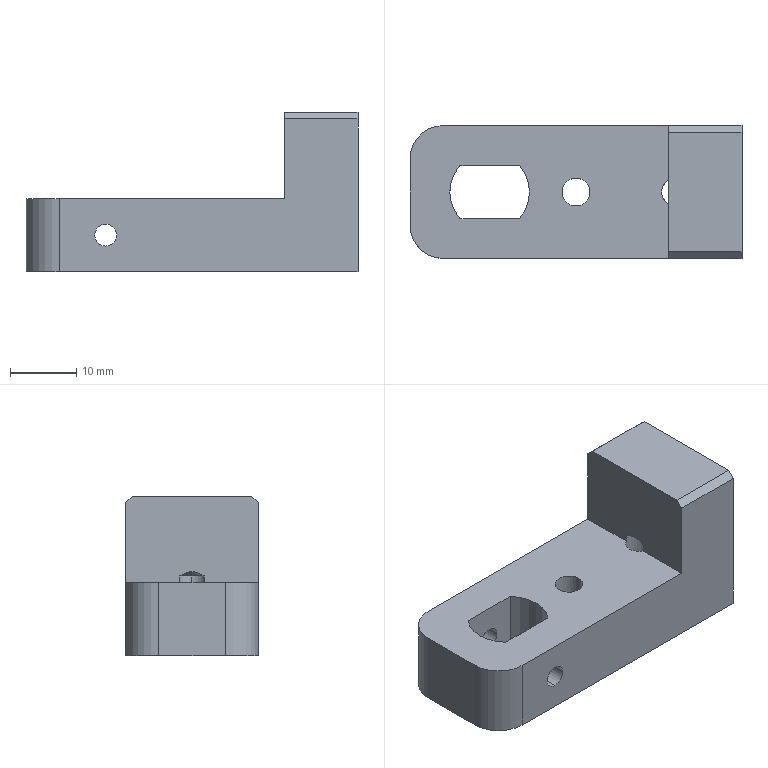Component | SolidWorks | TensioningWheel-2-1_XT-1-20-2-1 | 1 solid | 27 faces | box 50 x 20 x 24 mm | volume 12336 mm3 | cylinder 13 | plane 12 | cone 2 | commonest cylinder face diameters 3.3 x4 4.2 x4 12 x3 10 x2
build123d program:
from build123d import *

# Parameters (mm, degrees)
SKETCH1_W             = 50
SKETCH1_H             = 20
BOSS_EXTRUDE1_DEPTH   = 11
SKETCH7_W             = 11
SKETCH7_H             = 20
BOSS_EXTRUDE3_DEPTH   = 13
M5_TAPPED_HOLE1_D     = 4.2
M5_TAPPED_HOLE1_DEPTH = 12
M5_TAPPED_HOLE1_TIP   = 1.262
FILLET1_R             = 5
M4_TAPPED_HOLE1_D     = 3.3
CHAMFER1_SIZE         = 1


with BuildPart() as part:
    # Sketch1 → Boss-Extrude1 (new body)
    with BuildSketch(Plane.XY):
        with Locations((25, -10)):
            Rectangle(SKETCH1_W, SKETCH1_H)
        with BuildLine():
            Line((7.528, -6), (16.472, -6))
            ThreePointArc((16.472, -6), (18, -10), (16.472, -14))
            Line((16.472, -14), (7.528, -14))
            ThreePointArc((7.528, -14), (6, -10), (7.528, -6))
        make_face(mode=Mode.SUBTRACT)
    extrude(amount=BOSS_EXTRUDE1_DEPTH)

    # Sketch7 → Boss-Extrude3 (add)
    with BuildSketch(Plane.XY.offset(11)):
        with Locations((44.5, -10)):
            Rectangle(SKETCH7_W, SKETCH7_H)
    extrude(amount=BOSS_EXTRUDE3_DEPTH)

    # M5 Tapped Hole1
    with Locations(Plane(origin=(0, 0, 0), x_dir=(-1, 0, 0), z_dir=(0, 0, -1))):
        with Locations((-40, -10), (-25, -10)):
            Hole(M5_TAPPED_HOLE1_D / 2, depth=M5_TAPPED_HOLE1_DEPTH)
            with Locations((0, 0, -(M5_TAPPED_HOLE1_DEPTH + M5_TAPPED_HOLE1_TIP / 2))):  # 118° drill point
                Cone(0, M5_TAPPED_HOLE1_D / 2, M5_TAPPED_HOLE1_TIP, mode=Mode.SUBTRACT)

    # Fillet1
    fillet1_edges = [part.edges().sort_by_distance(p)[0] for p in [
        (0, -20, 5.5),
        (0, 0, 5.5),
    ]]
    fillet(fillet1_edges, radius=FILLET1_R)

    # M4 Tapped Hole1 (through all)
    with Locations(Plane(origin=(0, 0, 0), x_dir=(1, 0, 0), z_dir=(0, 1, 0))):
        with Locations((12, -5.5)):
            Hole(M4_TAPPED_HOLE1_D / 2)

    # Chamfer1
    chamfer1_edges = [part.edges().sort_by_distance(p)[0] for p in [
        (44.5, -20, 24),
        (44.5, 0, 24),
    ]]
    chamfer(chamfer1_edges, length=CHAMFER1_SIZE)


solid = part.part

# Placed as in the assembly
solid = solid.moved(Location((526.036, -108.615, -151), (0, 0, 0)))
STEP:
#1=CARTESIAN_POINT('',(21.183,-5.064,-5.793));
#2=VERTEX_POINT('',#1);
#3=CARTESIAN_POINT('',(21.183,-5.064,-5.663));
#4=VERTEX_POINT('',#3);
#5=CARTESIAN_POINT('',(21.183,-5.064,-5.728));
#6=DIRECTION('',(0.,1.,0.));
#7=DIRECTION('',(0.,0.,1.));
#8=AXIS2_PLACEMENT_3D('',#5,#6,#7);
#9=CIRCLE('',#8,0.06496);
#10=EDGE_CURVE('',#2,#4,#9,.T.);
#11=ORIENTED_EDGE('',*,*,#10,.F.);
#12=CARTESIAN_POINT('',(21.183,-4.827,-5.793));
#13=VERTEX_POINT('',#12);
#14=CARTESIAN_POINT('',(21.183,-4.276,-5.793));
#15=DIRECTION('',(0.,1.,0.));
#16=VECTOR('',#15,39.37);
#17=LINE('',#14,#16);
#18=EDGE_CURVE('',#2,#13,#17,.T.);
#19=ORIENTED_EDGE('',*,*,#18,.T.);
#20=CARTESIAN_POINT('',(21.183,-4.827,-5.663));
#21=VERTEX_POINT('',#20);
#22=CARTESIAN_POINT('',(21.183,-4.827,-5.728));
#23=DIRECTION('',(0.,1.,0.));
#24=DIRECTION('',(0.,0.,1.));
#25=AXIS2_PLACEMENT_3D('',#22,#23,#24);
#26=CIRCLE('',#25,0.06496);
#27=EDGE_CURVE('',#13,#21,#26,.T.);
#28=ORIENTED_EDGE('',*,*,#27,.T.);
#29=CARTESIAN_POINT('',(21.183,-4.276,-5.663));
#30=DIRECTION('',(0.,1.,0.));
#31=VECTOR('',#30,39.37);
#32=LINE('',#29,#31);
#33=EDGE_CURVE('',#4,#21,#32,.T.);
#34=ORIENTED_EDGE('',*,*,#33,.F.);
#35=EDGE_LOOP('',(#11,#19,#28,#34));
#36=FACE_OUTER_BOUND('',#35,.T.);
#37=CARTESIAN_POINT('',(21.183,-4.276,-5.728));
#38=DIRECTION('',(0.,1.,0.));
#39=DIRECTION('',(0.,0.,1.));
#40=AXIS2_PLACEMENT_3D('',#37,#38,#39);
#41=CYLINDRICAL_SURFACE('',#40,0.06496);
#42=ADVANCED_FACE('',(#36),#41,.F.);
#43=CARTESIAN_POINT('',(21.183,-4.512,-5.663));
#44=VERTEX_POINT('',#43);
#45=CARTESIAN_POINT('',(21.183,-4.512,-5.793));
#46=VERTEX_POINT('',#45);
#47=CARTESIAN_POINT('',(21.183,-4.512,-5.728));
#48=DIRECTION('',(0.,-1.,0.));
#49=DIRECTION('',(0.,0.,-1.));
#50=AXIS2_PLACEMENT_3D('',#47,#48,#49);
#51=CIRCLE('',#50,0.06496);
#52=EDGE_CURVE('',#44,#46,#51,.T.);
#53=ORIENTED_EDGE('',*,*,#52,.T.);
#54=CARTESIAN_POINT('',(21.183,-4.276,-5.793));
#55=VERTEX_POINT('',#54);
#56=CARTESIAN_POINT('',(21.183,-4.276,-5.793));
#57=DIRECTION('',(0.,1.,0.));
#58=VECTOR('',#57,39.37);
#59=LINE('',#56,#58);
#60=EDGE_CURVE('',#46,#55,#59,.T.);
#61=ORIENTED_EDGE('',*,*,#60,.T.);
#62=CARTESIAN_POINT('',(21.183,-4.276,-5.663));
#63=VERTEX_POINT('',#62);
#64=CARTESIAN_POINT('',(21.183,-4.276,-5.728));
#65=DIRECTION('',(0.,1.,0.));
#66=DIRECTION('',(0.,0.,1.));
#67=AXIS2_PLACEMENT_3D('',#64,#65,#66);
#68=CIRCLE('',#67,0.06496);
#69=EDGE_CURVE('',#55,#63,#68,.T.);
#70=ORIENTED_EDGE('',*,*,#69,.T.);
#71=CARTESIAN_POINT('',(21.183,-4.276,-5.663));
#72=DIRECTION('',(0.,1.,0.));
#73=VECTOR('',#72,39.37);
#74=LINE('',#71,#73);
#75=EDGE_CURVE('',#44,#63,#74,.T.);
#76=ORIENTED_EDGE('',*,*,#75,.F.);
#77=EDGE_LOOP('',(#53,#61,#70,#76));
#78=FACE_OUTER_BOUND('',#77,.T.);
#79=CARTESIAN_POINT('',(21.183,-4.276,-5.728));
#80=DIRECTION('',(0.,1.,0.));
#81=DIRECTION('',(0.,0.,1.));
#82=AXIS2_PLACEMENT_3D('',#79,#80,#81);
#83=CYLINDRICAL_SURFACE('',#82,0.06496);
#84=ADVANCED_FACE('',(#78),#83,.F.);
#85=CARTESIAN_POINT('',(22.285,-4.67,-5.423));
#86=VERTEX_POINT('',#85);
#87=CARTESIAN_POINT('',(22.246,-4.67,-5.446));
#88=VERTEX_POINT('',#87);
#89=CARTESIAN_POINT('',(22.202,-4.67,-5.472));
#90=DIRECTION('',(-0.8572,0.,-0.515));
#91=VECTOR('',#90,39.37);
#92=LINE('',#89,#91);
#93=EDGE_CURVE('',#86,#88,#92,.T.);
#94=ORIENTED_EDGE('',*,*,#93,.F.);
#95=CARTESIAN_POINT('',(22.368,-4.67,-5.472));
#96=VERTEX_POINT('',#95);
#97=CARTESIAN_POINT('',(22.368,-4.67,-5.472));
#98=DIRECTION('',(0.8572,0.,-0.515));
#99=VECTOR('',#98,39.37);
#100=LINE('',#97,#99);
#101=EDGE_CURVE('',#86,#96,#100,.T.);
#102=ORIENTED_EDGE('',*,*,#101,.T.);
#103=CARTESIAN_POINT('',(22.246,-4.743,-5.472));
#104=VERTEX_POINT('',#103);
#105=CARTESIAN_POINT('',(22.285,-4.67,-5.472));
#106=DIRECTION('',(0.,0.,-1.));
#107=DIRECTION('',(-1.,0.,0.));
#108=AXIS2_PLACEMENT_3D('',#105,#106,#107);
#109=CIRCLE('',#108,0.08268);
#110=EDGE_CURVE('',#96,#104,#109,.T.);
#111=ORIENTED_EDGE('',*,*,#110,.T.);
#112=CARTESIAN_POINT('',(22.246,-4.67,-5.446));
#113=CARTESIAN_POINT('',(22.246,-4.683,-5.446));
#114=CARTESIAN_POINT('',(22.246,-4.696,-5.451));
#115=CARTESIAN_POINT('',(22.246,-4.72,-5.46));
#116=CARTESIAN_POINT('',(22.246,-4.731,-5.466));
#117=CARTESIAN_POINT('',(22.246,-4.743,-5.472));
#118=B_SPLINE_CURVE_WITH_KNOTS('',3,(#112,#113,#114,#115,#116,#117),.UNSPECIFIED.,.F.,.F.,(4,2,4),(0.001979,0.002973,0.003966),.UNSPECIFIED.);
#119=EDGE_CURVE('',#88,#104,#118,.T.);
#120=ORIENTED_EDGE('',*,*,#119,.F.);
#121=EDGE_LOOP('',(#94,#102,#111,#120));
#122=FACE_OUTER_BOUND('',#121,.T.);
#123=CARTESIAN_POINT('',(22.285,-4.67,-5.472));
#124=DIRECTION('',(0.,0.,-1.));
#125=DIRECTION('',(-1.,0.,0.));
#126=AXIS2_PLACEMENT_3D('',#123,#124,#125);
#127=CONICAL_SURFACE('',#126,0.08268,1.03);
#128=ADVANCED_FACE('',(#122),#127,.F.);
#129=ORIENTED_EDGE('',*,*,#110,.F.);
#130=CARTESIAN_POINT('',(22.368,-4.67,-5.945));
#131=VERTEX_POINT('',#130);
#132=CARTESIAN_POINT('',(22.368,-4.67,-5.945));
#133=DIRECTION('',(0.,0.,-1.));
#134=VECTOR('',#133,39.37);
#135=LINE('',#132,#134);
#136=EDGE_CURVE('',#96,#131,#135,.T.);
#137=ORIENTED_EDGE('',*,*,#136,.T.);
#138=CARTESIAN_POINT('',(22.202,-4.67,-5.945));
#139=VERTEX_POINT('',#138);
#140=CARTESIAN_POINT('',(22.285,-4.67,-5.945));
#141=DIRECTION('',(0.,0.,-1.));
#142=DIRECTION('',(-1.,0.,0.));
#143=AXIS2_PLACEMENT_3D('',#140,#141,#142);
#144=CIRCLE('',#143,0.08268);
#145=EDGE_CURVE('',#131,#139,#144,.T.);
#146=ORIENTED_EDGE('',*,*,#145,.T.);
#147=CARTESIAN_POINT('',(22.202,-4.67,-5.512));
#148=VERTEX_POINT('',#147);
#149=CARTESIAN_POINT('',(22.202,-4.67,-5.945));
#150=DIRECTION('',(0.,0.,-1.));
#151=VECTOR('',#150,39.37);
#152=LINE('',#149,#151);
#153=EDGE_CURVE('',#148,#139,#152,.T.);
#154=ORIENTED_EDGE('',*,*,#153,.F.);
#155=CARTESIAN_POINT('',(22.246,-4.743,-5.512));
#156=VERTEX_POINT('',#155);
#157=CARTESIAN_POINT('',(22.285,-4.67,-5.512));
#158=DIRECTION('',(0.,0.,1.));
#159=DIRECTION('',(1.,0.,0.));
#160=AXIS2_PLACEMENT_3D('',#157,#158,#159);
#161=CIRCLE('',#160,0.08268);
#162=EDGE_CURVE('',#148,#156,#161,.T.);
#163=ORIENTED_EDGE('',*,*,#162,.T.);
#164=CARTESIAN_POINT('',(22.246,-4.743,-5.945));
#165=DIRECTION('',(0.,0.,-1.));
#166=VECTOR('',#165,39.37);
#167=LINE('',#164,#166);
#168=EDGE_CURVE('',#104,#156,#167,.T.);
#169=ORIENTED_EDGE('',*,*,#168,.F.);
#170=EDGE_LOOP('',(#129,#137,#146,#154,#163,#169));
#171=FACE_OUTER_BOUND('',#170,.T.);
#172=CARTESIAN_POINT('',(22.285,-4.67,-5.945));
#173=DIRECTION('',(0.,0.,-1.));
#174=DIRECTION('',(-1.,0.,0.));
#175=AXIS2_PLACEMENT_3D('',#172,#173,#174);
#176=CYLINDRICAL_SURFACE('',#175,0.08268);
#177=ADVANCED_FACE('',(#171),#176,.F.);
#178=CARTESIAN_POINT('',(21.612,-4.67,-5.512));
#179=VERTEX_POINT('',#178);
#180=CARTESIAN_POINT('',(21.777,-4.67,-5.512));
#181=VERTEX_POINT('',#180);
#182=CARTESIAN_POINT('',(21.694,-4.67,-5.512));
#183=DIRECTION('',(0.,0.,1.));
#184=DIRECTION('',(1.,0.,0.));
#185=AXIS2_PLACEMENT_3D('',#182,#183,#184);
#186=CIRCLE('',#185,0.08268);
#187=EDGE_CURVE('',#179,#181,#186,.T.);
#188=ORIENTED_EDGE('',*,*,#187,.T.);
#189=CARTESIAN_POINT('',(21.777,-4.67,-5.945));
#190=VERTEX_POINT('',#189);
#191=CARTESIAN_POINT('',(21.777,-4.67,-5.945));
#192=DIRECTION('',(0.,0.,-1.));
#193=VECTOR('',#192,39.37);
#194=LINE('',#191,#193);
#195=EDGE_CURVE('',#181,#190,#194,.T.);
#196=ORIENTED_EDGE('',*,*,#195,.T.);
#197=CARTESIAN_POINT('',(21.612,-4.67,-5.945));
#198=VERTEX_POINT('',#197);
#199=CARTESIAN_POINT('',(21.694,-4.67,-5.945));
#200=DIRECTION('',(0.,0.,-1.));
#201=DIRECTION('',(-1.,0.,0.));
#202=AXIS2_PLACEMENT_3D('',#199,#200,#201);
#203=CIRCLE('',#202,0.08268);
#204=EDGE_CURVE('',#190,#198,#203,.T.);
#205=ORIENTED_EDGE('',*,*,#204,.T.);
#206=CARTESIAN_POINT('',(21.612,-4.67,-5.945));
#207=DIRECTION('',(0.,0.,-1.));
#208=VECTOR('',#207,39.37);
#209=LINE('',#206,#208);
#210=EDGE_CURVE('',#179,#198,#209,.T.);
#211=ORIENTED_EDGE('',*,*,#210,.F.);
#212=EDGE_LOOP('',(#188,#196,#205,#211));
#213=FACE_OUTER_BOUND('',#212,.T.);
#214=CARTESIAN_POINT('',(21.694,-4.67,-5.945));
#215=DIRECTION('',(0.,0.,-1.));
#216=DIRECTION('',(-1.,0.,0.));
#217=AXIS2_PLACEMENT_3D('',#214,#215,#216);
#218=CYLINDRICAL_SURFACE('',#217,0.08268);
#219=ADVANCED_FACE('',(#213),#218,.F.);
#220=CARTESIAN_POINT('',(21.006,-4.512,-5.512));
#221=VERTEX_POINT('',#220);
#222=CARTESIAN_POINT('',(20.946,-4.67,-5.512));
#223=VERTEX_POINT('',#222);
#224=CARTESIAN_POINT('',(21.183,-4.67,-5.512));
#225=DIRECTION('',(0.,0.,1.));
#226=DIRECTION('',(1.,0.,0.));
#227=AXIS2_PLACEMENT_3D('',#224,#225,#226);
#228=CIRCLE('',#227,0.2362);
#229=EDGE_CURVE('',#221,#223,#228,.T.);
#230=ORIENTED_EDGE('',*,*,#229,.T.);
#231=CARTESIAN_POINT('',(20.946,-4.67,-5.945));
#232=VERTEX_POINT('',#231);
#233=CARTESIAN_POINT('',(20.946,-4.67,-5.512));
#234=DIRECTION('',(0.,0.,-1.));
#235=VECTOR('',#234,39.37);
#236=LINE('',#233,#235);
#237=EDGE_CURVE('',#223,#232,#236,.T.);
#238=ORIENTED_EDGE('',*,*,#237,.T.);
#239=CARTESIAN_POINT('',(21.006,-4.512,-5.945));
#240=VERTEX_POINT('',#239);
#241=CARTESIAN_POINT('',(21.183,-4.67,-5.945));
#242=DIRECTION('',(0.,0.,1.));
#243=DIRECTION('',(1.,0.,0.));
#244=AXIS2_PLACEMENT_3D('',#241,#242,#243);
#245=CIRCLE('',#244,0.2362);
#246=EDGE_CURVE('',#240,#232,#245,.T.);
#247=ORIENTED_EDGE('',*,*,#246,.F.);
#248=CARTESIAN_POINT('',(21.006,-4.512,-5.512));
#249=DIRECTION('',(0.,0.,-1.));
#250=VECTOR('',#249,39.37);
#251=LINE('',#248,#250);
#252=EDGE_CURVE('',#221,#240,#251,.T.);
#253=ORIENTED_EDGE('',*,*,#252,.F.);
#254=EDGE_LOOP('',(#230,#238,#247,#253));
#255=FACE_OUTER_BOUND('',#254,.T.);
#256=CARTESIAN_POINT('',(21.183,-4.67,-5.512));
#257=DIRECTION('',(0.,0.,-1.));
#258=DIRECTION('',(-1.,0.,0.));
#259=AXIS2_PLACEMENT_3D('',#256,#257,#258);
#260=CYLINDRICAL_SURFACE('',#259,0.2362);
#261=ADVANCED_FACE('',(#255),#260,.F.);
#262=CARTESIAN_POINT('',(20.71,-4.473,-5.512));
#263=VERTEX_POINT('',#262);
#264=CARTESIAN_POINT('',(20.71,-4.867,-5.512));
#265=VERTEX_POINT('',#264);
#266=CARTESIAN_POINT('',(20.71,-4.276,-5.512));
#267=DIRECTION('',(0.,-1.,0.));
#268=VECTOR('',#267,39.37);
#269=LINE('',#266,#268);
#270=EDGE_CURVE('',#263,#265,#269,.T.);
#271=ORIENTED_EDGE('',*,*,#270,.T.);
#272=CARTESIAN_POINT('',(20.907,-5.064,-5.512));
#273=VERTEX_POINT('',#272);
#274=CARTESIAN_POINT('',(20.907,-4.867,-5.512));
#275=DIRECTION('',(0.,0.,1.));
#276=DIRECTION('',(1.,0.,0.));
#277=AXIS2_PLACEMENT_3D('',#274,#275,#276);
#278=CIRCLE('',#277,0.1969);
#279=EDGE_CURVE('',#265,#273,#278,.T.);
#280=ORIENTED_EDGE('',*,*,#279,.T.);
#281=CARTESIAN_POINT('',(22.246,-5.064,-5.512));
#282=VERTEX_POINT('',#281);
#283=CARTESIAN_POINT('',(20.71,-5.064,-5.512));
#284=DIRECTION('',(1.,0.,0.));
#285=VECTOR('',#284,39.37);
#286=LINE('',#283,#285);
#287=EDGE_CURVE('',#273,#282,#286,.T.);
#288=ORIENTED_EDGE('',*,*,#287,.T.);
#289=CARTESIAN_POINT('',(22.246,-4.276,-5.512));
#290=DIRECTION('',(0.,-1.,0.));
#291=VECTOR('',#290,39.37);
#292=LINE('',#289,#291);
#293=EDGE_CURVE('',#156,#282,#292,.T.);
#294=ORIENTED_EDGE('',*,*,#293,.F.);
#295=ORIENTED_EDGE('',*,*,#162,.F.);
#296=CARTESIAN_POINT('',(22.246,-4.597,-5.512));
#297=VERTEX_POINT('',#296);
#298=CARTESIAN_POINT('',(22.285,-4.67,-5.512));
#299=DIRECTION('',(0.,0.,1.));
#300=DIRECTION('',(1.,0.,0.));
#301=AXIS2_PLACEMENT_3D('',#298,#299,#300);
#302=CIRCLE('',#301,0.08268);
#303=EDGE_CURVE('',#297,#148,#302,.T.);
#304=ORIENTED_EDGE('',*,*,#303,.F.);
#305=CARTESIAN_POINT('',(22.246,-4.276,-5.512));
#306=VERTEX_POINT('',#305);
#307=CARTESIAN_POINT('',(22.246,-4.276,-5.512));
#308=DIRECTION('',(0.,-1.,0.));
#309=VECTOR('',#308,39.37);
#310=LINE('',#307,#309);
#311=EDGE_CURVE('',#306,#297,#310,.T.);
#312=ORIENTED_EDGE('',*,*,#311,.F.);
#313=CARTESIAN_POINT('',(20.907,-4.276,-5.512));
#314=VERTEX_POINT('',#313);
#315=CARTESIAN_POINT('',(20.71,-4.276,-5.512));
#316=DIRECTION('',(-1.,0.,0.));
#317=VECTOR('',#316,39.37);
#318=LINE('',#315,#317);
#319=EDGE_CURVE('',#306,#314,#318,.T.);
#320=ORIENTED_EDGE('',*,*,#319,.T.);
#321=CARTESIAN_POINT('',(20.907,-4.473,-5.512));
#322=DIRECTION('',(0.,0.,1.));
#323=DIRECTION('',(1.,0.,0.));
#324=AXIS2_PLACEMENT_3D('',#321,#322,#323);
#325=CIRCLE('',#324,0.1969);
#326=EDGE_CURVE('',#314,#263,#325,.T.);
#327=ORIENTED_EDGE('',*,*,#326,.T.);
#328=EDGE_LOOP('',(#271,#280,#288,#294,#295,#304,#312,#320,#327));
#329=FACE_OUTER_BOUND('',#328,.T.);
#330=ORIENTED_EDGE('',*,*,#187,.F.);
#331=CARTESIAN_POINT('',(21.694,-4.67,-5.512));
#332=DIRECTION('',(0.,0.,1.));
#333=DIRECTION('',(1.,0.,0.));
#334=AXIS2_PLACEMENT_3D('',#331,#332,#333);
#335=CIRCLE('',#334,0.08268);
#336=EDGE_CURVE('',#181,#179,#335,.T.);
#337=ORIENTED_EDGE('',*,*,#336,.F.);
#338=EDGE_LOOP('',(#330,#337));
#339=FACE_BOUND('',#338,.T.);
#340=CARTESIAN_POINT('',(21.006,-4.827,-5.512));
#341=VERTEX_POINT('',#340);
#342=CARTESIAN_POINT('',(21.359,-4.827,-5.512));
#343=VERTEX_POINT('',#342);
#344=CARTESIAN_POINT('',(21.006,-4.827,-5.512));
#345=DIRECTION('',(1.,0.,0.));
#346=VECTOR('',#345,39.37);
#347=LINE('',#344,#346);
#348=EDGE_CURVE('',#341,#343,#347,.T.);
#349=ORIENTED_EDGE('',*,*,#348,.F.);
#350=CARTESIAN_POINT('',(21.183,-4.67,-5.512));
#351=DIRECTION('',(0.,0.,1.));
#352=DIRECTION('',(1.,0.,0.));
#353=AXIS2_PLACEMENT_3D('',#350,#351,#352);
#354=CIRCLE('',#353,0.2362);
#355=EDGE_CURVE('',#223,#341,#354,.T.);
#356=ORIENTED_EDGE('',*,*,#355,.F.);
#357=ORIENTED_EDGE('',*,*,#229,.F.);
#358=CARTESIAN_POINT('',(21.359,-4.512,-5.512));
#359=VERTEX_POINT('',#358);
#360=CARTESIAN_POINT('',(21.006,-4.512,-5.512));
#361=DIRECTION('',(-1.,0.,0.));
#362=VECTOR('',#361,39.37);
#363=LINE('',#360,#362);
#364=EDGE_CURVE('',#359,#221,#363,.T.);
#365=ORIENTED_EDGE('',*,*,#364,.F.);
#366=CARTESIAN_POINT('',(21.183,-4.67,-5.512));
#367=DIRECTION('',(0.,0.,1.));
#368=DIRECTION('',(1.,0.,0.));
#369=AXIS2_PLACEMENT_3D('',#366,#367,#368);
#370=CIRCLE('',#369,0.2362);
#371=EDGE_CURVE('',#343,#359,#370,.T.);
#372=ORIENTED_EDGE('',*,*,#371,.F.);
#373=EDGE_LOOP('',(#349,#356,#357,#365,#372));
#374=FACE_BOUND('',#373,.T.);
#375=CARTESIAN_POINT('',(20.71,-4.276,-5.512));
#376=DIRECTION('',(0.,0.,1.));
#377=DIRECTION('',(1.,0.,0.));
#378=AXIS2_PLACEMENT_3D('',#375,#376,#377);
#379=PLANE('',#378);
#380=ADVANCED_FACE('',(#329,#339,#374),#379,.T.);
#381=CARTESIAN_POINT('',(22.285,-4.67,-5.945));
#382=DIRECTION('',(0.,0.,-1.));
#383=DIRECTION('',(-1.,0.,0.));
#384=AXIS2_PLACEMENT_3D('',#381,#382,#383);
#385=CIRCLE('',#384,0.08268);
#386=EDGE_CURVE('',#139,#131,#385,.T.);
#387=ORIENTED_EDGE('',*,*,#386,.F.);
#388=ORIENTED_EDGE('',*,*,#145,.F.);
#389=EDGE_LOOP('',(#387,#388));
#390=FACE_BOUND('',#389,.T.);
#391=CARTESIAN_POINT('',(21.694,-4.67,-5.945));
#392=DIRECTION('',(0.,0.,-1.));
#393=DIRECTION('',(-1.,0.,0.));
#394=AXIS2_PLACEMENT_3D('',#391,#392,#393);
#395=CIRCLE('',#394,0.08268);
#396=EDGE_CURVE('',#198,#190,#395,.T.);
#397=ORIENTED_EDGE('',*,*,#396,.F.);
#398=ORIENTED_EDGE('',*,*,#204,.F.);
#399=EDGE_LOOP('',(#397,#398));
#400=FACE_BOUND('',#399,.T.);
#401=CARTESIAN_POINT('',(20.907,-5.064,-5.945));
#402=VERTEX_POINT('',#401);
#403=CARTESIAN_POINT('',(22.679,-5.064,-5.945));
#404=VERTEX_POINT('',#403);
#405=CARTESIAN_POINT('',(20.71,-5.064,-5.945));
#406=DIRECTION('',(1.,0.,0.));
#407=VECTOR('',#406,39.37);
#408=LINE('',#405,#407);
#409=EDGE_CURVE('',#402,#404,#408,.T.);
#410=ORIENTED_EDGE('',*,*,#409,.F.);
#411=CARTESIAN_POINT('',(20.71,-4.867,-5.945));
#412=VERTEX_POINT('',#411);
#413=CARTESIAN_POINT('',(20.907,-4.867,-5.945));
#414=DIRECTION('',(0.,0.,-1.));
#415=DIRECTION('',(1.,0.,0.));
#416=AXIS2_PLACEMENT_3D('',#413,#414,#415);
#417=CIRCLE('',#416,0.1969);
#418=EDGE_CURVE('',#402,#412,#417,.T.);
#419=ORIENTED_EDGE('',*,*,#418,.T.);
#420=CARTESIAN_POINT('',(20.71,-4.473,-5.945));
#421=VERTEX_POINT('',#420);
#422=CARTESIAN_POINT('',(20.71,-4.276,-5.945));
#423=DIRECTION('',(0.,-1.,0.));
#424=VECTOR('',#423,39.37);
#425=LINE('',#422,#424);
#426=EDGE_CURVE('',#421,#412,#425,.T.);
#427=ORIENTED_EDGE('',*,*,#426,.F.);
#428=CARTESIAN_POINT('',(20.907,-4.276,-5.945));
#429=VERTEX_POINT('',#428);
#430=CARTESIAN_POINT('',(20.907,-4.473,-5.945));
#431=DIRECTION('',(0.,0.,-1.));
#432=DIRECTION('',(1.,0.,0.));
#433=AXIS2_PLACEMENT_3D('',#430,#431,#432);
#434=CIRCLE('',#433,0.1969);
#435=EDGE_CURVE('',#421,#429,#434,.T.);
#436=ORIENTED_EDGE('',*,*,#435,.T.);
#437=CARTESIAN_POINT('',(22.679,-4.276,-5.945));
#438=VERTEX_POINT('',#437);
#439=CARTESIAN_POINT('',(20.71,-4.276,-5.945));
#440=DIRECTION('',(-1.,0.,0.));
#441=VECTOR('',#440,39.37);
#442=LINE('',#439,#441);
#443=EDGE_CURVE('',#438,#429,#442,.T.);
#444=ORIENTED_EDGE('',*,*,#443,.F.);
#445=CARTESIAN_POINT('',(22.679,-4.276,-5.945));
#446=DIRECTION('',(0.,1.,0.));
#447=VECTOR('',#446,39.37);
#448=LINE('',#445,#447);
#449=EDGE_CURVE('',#404,#438,#448,.T.);
#450=ORIENTED_EDGE('',*,*,#449,.F.);
#451=EDGE_LOOP('',(#410,#419,#427,#436,#444,#450));
#452=FACE_OUTER_BOUND('',#451,.T.);
#453=ORIENTED_EDGE('',*,*,#246,.T.);
#454=CARTESIAN_POINT('',(21.006,-4.827,-5.945));
#455=VERTEX_POINT('',#454);
#456=CARTESIAN_POINT('',(21.183,-4.67,-5.945));
#457=DIRECTION('',(0.,0.,1.));
#458=DIRECTION('',(1.,0.,0.));
#459=AXIS2_PLACEMENT_3D('',#456,#457,#458);
#460=CIRCLE('',#459,0.2362);
#461=EDGE_CURVE('',#232,#455,#460,.T.);
#462=ORIENTED_EDGE('',*,*,#461,.T.);
#463=CARTESIAN_POINT('',(21.359,-4.827,-5.945));
#464=VERTEX_POINT('',#463);
#465=CARTESIAN_POINT('',(21.006,-4.827,-5.945));
#466=DIRECTION('',(1.,0.,0.));
#467=VECTOR('',#466,39.37);
#468=LINE('',#465,#467);
#469=EDGE_CURVE('',#455,#464,#468,.T.);
#470=ORIENTED_EDGE('',*,*,#469,.T.);
#471=CARTESIAN_POINT('',(21.359,-4.512,-5.945));
#472=VERTEX_POINT('',#471);
#473=CARTESIAN_POINT('',(21.183,-4.67,-5.945));
#474=DIRECTION('',(0.,0.,1.));
#475=DIRECTION('',(1.,0.,0.));
#476=AXIS2_PLACEMENT_3D('',#473,#474,#475);
#477=CIRCLE('',#476,0.2362);
#478=EDGE_CURVE('',#464,#472,#477,.T.);
#479=ORIENTED_EDGE('',*,*,#478,.T.);
#480=CARTESIAN_POINT('',(21.006,-4.512,-5.945));
#481=DIRECTION('',(-1.,0.,0.));
#482=VECTOR('',#481,39.37);
#483=LINE('',#480,#482);
#484=EDGE_CURVE('',#472,#240,#483,.T.);
#485=ORIENTED_EDGE('',*,*,#484,.T.);
#486=EDGE_LOOP('',(#453,#462,#470,#479,#485));
#487=FACE_BOUND('',#486,.T.);
#488=CARTESIAN_POINT('',(20.71,-4.276,-5.945));
#489=DIRECTION('',(0.,0.,1.));
#490=DIRECTION('',(1.,0.,0.));
#491=AXIS2_PLACEMENT_3D('',#488,#489,#490);
#492=PLANE('',#491);
#493=ADVANCED_FACE('',(#390,#400,#452,#487),#492,.F.);
#494=ORIENTED_EDGE('',*,*,#426,.T.);
#495=CARTESIAN_POINT('',(20.71,-4.867,-5.512));
#496=DIRECTION('',(0.,0.,1.));
#497=VECTOR('',#496,39.37);
#498=LINE('',#495,#497);
#499=EDGE_CURVE('',#412,#265,#498,.T.);
#500=ORIENTED_EDGE('',*,*,#499,.T.);
#501=ORIENTED_EDGE('',*,*,#270,.F.);
#502=CARTESIAN_POINT('',(20.71,-4.473,-5.512));
#503=DIRECTION('',(0.,0.,-1.));
#504=VECTOR('',#503,39.37);
#505=LINE('',#502,#504);
#506=EDGE_CURVE('',#263,#421,#505,.T.);
#507=ORIENTED_EDGE('',*,*,#506,.T.);
#508=EDGE_LOOP('',(#494,#500,#501,#507));
#509=FACE_OUTER_BOUND('',#508,.T.);
#510=CARTESIAN_POINT('',(20.71,-4.276,-5.512));
#511=DIRECTION('',(1.,0.,0.));
#512=DIRECTION('',(-0.,1.,0.));
#513=AXIS2_PLACEMENT_3D('',#510,#511,#512);
#514=PLANE('',#513);
#515=ADVANCED_FACE('',(#509),#514,.F.);
#516=CARTESIAN_POINT('',(21.183,-5.064,-5.728));
#517=DIRECTION('',(0.,1.,0.));
#518=DIRECTION('',(0.,0.,1.));
#519=AXIS2_PLACEMENT_3D('',#516,#517,#518);
#520=CIRCLE('',#519,0.06496);
#521=EDGE_CURVE('',#4,#2,#520,.T.);
#522=ORIENTED_EDGE('',*,*,#521,.T.);
#523=ORIENTED_EDGE('',*,*,#10,.T.);
#524=EDGE_LOOP('',(#522,#523));
#525=FACE_BOUND('',#524,.T.);
#526=CARTESIAN_POINT('',(22.679,-5.064,-5.039));
#527=VERTEX_POINT('',#526);
#528=CARTESIAN_POINT('',(22.679,-5.064,-5.512));
#529=DIRECTION('',(0.,0.,-1.));
#530=VECTOR('',#529,39.37);
#531=LINE('',#528,#530);
#532=EDGE_CURVE('',#527,#404,#531,.T.);
#533=ORIENTED_EDGE('',*,*,#532,.F.);
#534=CARTESIAN_POINT('',(22.246,-5.064,-5.039));
#535=VERTEX_POINT('',#534);
#536=CARTESIAN_POINT('',(20.71,-5.064,-5.039));
#537=DIRECTION('',(-1.,0.,0.));
#538=VECTOR('',#537,39.37);
#539=LINE('',#536,#538);
#540=EDGE_CURVE('',#527,#535,#539,.T.);
#541=ORIENTED_EDGE('',*,*,#540,.T.);
#542=CARTESIAN_POINT('',(22.246,-5.064,-5.));
#543=DIRECTION('',(0.,0.,-1.));
#544=VECTOR('',#543,39.37);
#545=LINE('',#542,#544);
#546=EDGE_CURVE('',#535,#282,#545,.T.);
#547=ORIENTED_EDGE('',*,*,#546,.T.);
#548=ORIENTED_EDGE('',*,*,#287,.F.);
#549=CARTESIAN_POINT('',(20.907,-5.064,-5.512));
#550=DIRECTION('',(0.,0.,-1.));
#551=VECTOR('',#550,39.37);
#552=LINE('',#549,#551);
#553=EDGE_CURVE('',#273,#402,#552,.T.);
#554=ORIENTED_EDGE('',*,*,#553,.T.);
#555=ORIENTED_EDGE('',*,*,#409,.T.);
#556=EDGE_LOOP('',(#533,#541,#547,#548,#554,#555));
#557=FACE_OUTER_BOUND('',#556,.T.);
#558=CARTESIAN_POINT('',(20.71,-5.064,-5.512));
#559=DIRECTION('',(0.,1.,0.));
#560=DIRECTION('',(0.,0.,1.));
#561=AXIS2_PLACEMENT_3D('',#558,#559,#560);
#562=PLANE('',#561);
#563=ADVANCED_FACE('',(#525,#557),#562,.F.);
#564=CARTESIAN_POINT('',(22.679,-5.024,-5.));
#565=VERTEX_POINT('',#564);
#566=CARTESIAN_POINT('',(22.679,-4.316,-5.));
#567=VERTEX_POINT('',#566);
#568=CARTESIAN_POINT('',(22.679,-4.276,-5.));
#569=DIRECTION('',(0.,1.,0.));
#570=VECTOR('',#569,39.37);
#571=LINE('',#568,#570);
#572=EDGE_CURVE('',#565,#567,#571,.T.);
#573=ORIENTED_EDGE('',*,*,#572,.F.);
#574=CARTESIAN_POINT('',(22.679,-5.024,-5.));
#575=DIRECTION('',(0.,-0.7071,-0.7071));
#576=VECTOR('',#575,39.37);
#577=LINE('',#574,#576);
#578=EDGE_CURVE('',#565,#527,#577,.T.);
#579=ORIENTED_EDGE('',*,*,#578,.T.);
#580=ORIENTED_EDGE('',*,*,#532,.T.);
#581=ORIENTED_EDGE('',*,*,#449,.T.);
#582=CARTESIAN_POINT('',(22.679,-4.276,-5.039));
#583=VERTEX_POINT('',#582);
#584=CARTESIAN_POINT('',(22.679,-4.276,-5.512));
#585=DIRECTION('',(0.,0.,-1.));
#586=VECTOR('',#585,39.37);
#587=LINE('',#584,#586);
#588=EDGE_CURVE('',#583,#438,#587,.T.);
#589=ORIENTED_EDGE('',*,*,#588,.F.);
#590=CARTESIAN_POINT('',(22.679,-4.316,-5.));
#591=DIRECTION('',(0.,-0.7071,0.7071));
#592=VECTOR('',#591,39.37);
#593=LINE('',#590,#592);
#594=EDGE_CURVE('',#583,#567,#593,.T.);
#595=ORIENTED_EDGE('',*,*,#594,.T.);
#596=EDGE_LOOP('',(#573,#579,#580,#581,#589,#595));
#597=FACE_OUTER_BOUND('',#596,.T.);
#598=CARTESIAN_POINT('',(22.679,-4.276,-5.512));
#599=DIRECTION('',(-1.,0.,0.));
#600=DIRECTION('',(0.,0.,1.));
#601=AXIS2_PLACEMENT_3D('',#598,#599,#600);
#602=PLANE('',#601);
#603=ADVANCED_FACE('',(#597),#602,.F.);
#604=CARTESIAN_POINT('',(21.183,-4.276,-5.728));
#605=DIRECTION('',(0.,1.,0.));
#606=DIRECTION('',(0.,0.,1.));
#607=AXIS2_PLACEMENT_3D('',#604,#605,#606);
#608=CIRCLE('',#607,0.06496);
#609=EDGE_CURVE('',#63,#55,#608,.T.);
#610=ORIENTED_EDGE('',*,*,#609,.F.);
#611=ORIENTED_EDGE('',*,*,#69,.F.);
#612=EDGE_LOOP('',(#610,#611));
#613=FACE_BOUND('',#612,.T.);
#614=CARTESIAN_POINT('',(22.246,-4.276,-5.039));
#615=VERTEX_POINT('',#614);
#616=CARTESIAN_POINT('',(22.246,-4.276,-5.));
#617=DIRECTION('',(0.,0.,-1.));
#618=VECTOR('',#617,39.37);
#619=LINE('',#616,#618);
#620=EDGE_CURVE('',#615,#306,#619,.T.);
#621=ORIENTED_EDGE('',*,*,#620,.F.);
#622=CARTESIAN_POINT('',(20.71,-4.276,-5.039));
#623=DIRECTION('',(1.,0.,0.));
#624=VECTOR('',#623,39.37);
#625=LINE('',#622,#624);
#626=EDGE_CURVE('',#615,#583,#625,.T.);
#627=ORIENTED_EDGE('',*,*,#626,.T.);
#628=ORIENTED_EDGE('',*,*,#588,.T.);
#629=ORIENTED_EDGE('',*,*,#443,.T.);
#630=CARTESIAN_POINT('',(20.907,-4.276,-5.512));
#631=DIRECTION('',(0.,0.,1.));
#632=VECTOR('',#631,39.37);
#633=LINE('',#630,#632);
#634=EDGE_CURVE('',#429,#314,#633,.T.);
#635=ORIENTED_EDGE('',*,*,#634,.T.);
#636=ORIENTED_EDGE('',*,*,#319,.F.);
#637=EDGE_LOOP('',(#621,#627,#628,#629,#635,#636));
#638=FACE_OUTER_BOUND('',#637,.T.);
#639=CARTESIAN_POINT('',(20.71,-4.276,-5.512));
#640=DIRECTION('',(0.,-1.,0.));
#641=DIRECTION('',(0.,0.,-1.));
#642=AXIS2_PLACEMENT_3D('',#639,#640,#641);
#643=PLANE('',#642);
#644=ADVANCED_FACE('',(#613,#638),#643,.F.);
#645=ORIENTED_EDGE('',*,*,#237,.F.);
#646=ORIENTED_EDGE('',*,*,#355,.T.);
#647=CARTESIAN_POINT('',(21.006,-4.827,-5.512));
#648=DIRECTION('',(0.,0.,-1.));
#649=VECTOR('',#648,39.37);
#650=LINE('',#647,#649);
#651=EDGE_CURVE('',#341,#455,#650,.T.);
#652=ORIENTED_EDGE('',*,*,#651,.T.);
#653=ORIENTED_EDGE('',*,*,#461,.F.);
#654=EDGE_LOOP('',(#645,#646,#652,#653));
#655=FACE_OUTER_BOUND('',#654,.T.);
#656=CARTESIAN_POINT('',(21.183,-4.67,-5.512));
#657=DIRECTION('',(0.,0.,-1.));
#658=DIRECTION('',(-1.,0.,0.));
#659=AXIS2_PLACEMENT_3D('',#656,#657,#658);
#660=CYLINDRICAL_SURFACE('',#659,0.2362);
#661=ADVANCED_FACE('',(#655),#660,.F.);
#662=CARTESIAN_POINT('',(21.183,-4.827,-5.728));
#663=DIRECTION('',(0.,1.,0.));
#664=DIRECTION('',(0.,0.,1.));
#665=AXIS2_PLACEMENT_3D('',#662,#663,#664);
#666=CIRCLE('',#665,0.06496);
#667=EDGE_CURVE('',#21,#13,#666,.T.);
#668=ORIENTED_EDGE('',*,*,#667,.F.);
#669=ORIENTED_EDGE('',*,*,#27,.F.);
#670=EDGE_LOOP('',(#668,#669));
#671=FACE_BOUND('',#670,.T.);
#672=ORIENTED_EDGE('',*,*,#469,.F.);
#673=ORIENTED_EDGE('',*,*,#651,.F.);
#674=ORIENTED_EDGE('',*,*,#348,.T.);
#675=CARTESIAN_POINT('',(21.359,-4.827,-5.512));
#676=DIRECTION('',(0.,0.,-1.));
#677=VECTOR('',#676,39.37);
#678=LINE('',#675,#677);
#679=EDGE_CURVE('',#343,#464,#678,.T.);
#680=ORIENTED_EDGE('',*,*,#679,.T.);
#681=EDGE_LOOP('',(#672,#673,#674,#680));
#682=FACE_OUTER_BOUND('',#681,.T.);
#683=CARTESIAN_POINT('',(21.006,-4.827,-5.512));
#684=DIRECTION('',(0.,1.,0.));
#685=DIRECTION('',(0.,0.,1.));
#686=AXIS2_PLACEMENT_3D('',#683,#684,#685);
#687=PLANE('',#686);
#688=ADVANCED_FACE('',(#671,#682),#687,.T.);
#689=ORIENTED_EDGE('',*,*,#478,.F.);
#690=ORIENTED_EDGE('',*,*,#679,.F.);
#691=ORIENTED_EDGE('',*,*,#371,.T.);
#692=CARTESIAN_POINT('',(21.359,-4.512,-5.512));
#693=DIRECTION('',(0.,0.,-1.));
#694=VECTOR('',#693,39.37);
#695=LINE('',#692,#694);
#696=EDGE_CURVE('',#359,#472,#695,.T.);
#697=ORIENTED_EDGE('',*,*,#696,.T.);
#698=EDGE_LOOP('',(#689,#690,#691,#697));
#699=FACE_OUTER_BOUND('',#698,.T.);
#700=CARTESIAN_POINT('',(21.183,-4.67,-5.512));
#701=DIRECTION('',(0.,0.,-1.));
#702=DIRECTION('',(-1.,0.,0.));
#703=AXIS2_PLACEMENT_3D('',#700,#701,#702);
#704=CYLINDRICAL_SURFACE('',#703,0.2362);
#705=ADVANCED_FACE('',(#699),#704,.F.);
#706=ORIENTED_EDGE('',*,*,#52,.F.);
#707=CARTESIAN_POINT('',(21.183,-4.512,-5.728));
#708=DIRECTION('',(0.,-1.,0.));
#709=DIRECTION('',(0.,0.,-1.));
#710=AXIS2_PLACEMENT_3D('',#707,#708,#709);
#711=CIRCLE('',#710,0.06496);
#712=EDGE_CURVE('',#46,#44,#711,.T.);
#713=ORIENTED_EDGE('',*,*,#712,.F.);
#714=EDGE_LOOP('',(#706,#713));
#715=FACE_BOUND('',#714,.T.);
#716=ORIENTED_EDGE('',*,*,#484,.F.);
#717=ORIENTED_EDGE('',*,*,#696,.F.);
#718=ORIENTED_EDGE('',*,*,#364,.T.);
#719=ORIENTED_EDGE('',*,*,#252,.T.);
#720=EDGE_LOOP('',(#716,#717,#718,#719));
#721=FACE_OUTER_BOUND('',#720,.T.);
#722=CARTESIAN_POINT('',(21.006,-4.512,-5.512));
#723=DIRECTION('',(0.,-1.,0.));
#724=DIRECTION('',(0.,0.,-1.));
#725=AXIS2_PLACEMENT_3D('',#722,#723,#724);
#726=PLANE('',#725);
#727=ADVANCED_FACE('',(#715,#721),#726,.T.);
#728=ORIENTED_EDGE('',*,*,#546,.F.);
#729=CARTESIAN_POINT('',(22.246,-5.024,-5.));
#730=VERTEX_POINT('',#729);
#731=CARTESIAN_POINT('',(22.246,-5.024,-5.));
#732=DIRECTION('',(0.,0.7071,0.7071));
#733=VECTOR('',#732,39.37);
#734=LINE('',#731,#733);
#735=EDGE_CURVE('',#535,#730,#734,.T.);
#736=ORIENTED_EDGE('',*,*,#735,.T.);
#737=CARTESIAN_POINT('',(22.246,-4.316,-5.));
#738=VERTEX_POINT('',#737);
#739=CARTESIAN_POINT('',(22.246,-4.276,-5.));
#740=DIRECTION('',(0.,-1.,0.));
#741=VECTOR('',#740,39.37);
#742=LINE('',#739,#741);
#743=EDGE_CURVE('',#738,#730,#742,.T.);
#744=ORIENTED_EDGE('',*,*,#743,.F.);
#745=CARTESIAN_POINT('',(22.246,-4.316,-5.));
#746=DIRECTION('',(0.,0.7071,-0.7071));
#747=VECTOR('',#746,39.37);
#748=LINE('',#745,#747);
#749=EDGE_CURVE('',#738,#615,#748,.T.);
#750=ORIENTED_EDGE('',*,*,#749,.T.);
#751=ORIENTED_EDGE('',*,*,#620,.T.);
#752=ORIENTED_EDGE('',*,*,#311,.T.);
#753=CARTESIAN_POINT('',(22.246,-4.597,-5.472));
#754=VERTEX_POINT('',#753);
#755=CARTESIAN_POINT('',(22.246,-4.597,-5.945));
#756=DIRECTION('',(0.,0.,1.));
#757=VECTOR('',#756,39.37);
#758=LINE('',#755,#757);
#759=EDGE_CURVE('',#297,#754,#758,.T.);
#760=ORIENTED_EDGE('',*,*,#759,.T.);
#761=CARTESIAN_POINT('',(22.246,-4.597,-5.472));
#762=CARTESIAN_POINT('',(22.246,-4.609,-5.466));
#763=CARTESIAN_POINT('',(22.246,-4.62,-5.46));
#764=CARTESIAN_POINT('',(22.246,-4.638,-5.453));
#765=CARTESIAN_POINT('',(22.246,-4.644,-5.451));
#766=CARTESIAN_POINT('',(22.246,-4.657,-5.447));
#767=CARTESIAN_POINT('',(22.246,-4.663,-5.446));
#768=CARTESIAN_POINT('',(22.246,-4.67,-5.446));
#769=B_SPLINE_CURVE_WITH_KNOTS('',3,(#761,#762,#763,#764,#765,#766,#767,#768),.UNSPECIFIED.,.F.,.F.,(4,2,2,4),(0.00000043,0.0009899,0.001485,0.001979),.UNSPECIFIED.);
#770=EDGE_CURVE('',#754,#88,#769,.T.);
#771=ORIENTED_EDGE('',*,*,#770,.T.);
#772=ORIENTED_EDGE('',*,*,#119,.T.);
#773=ORIENTED_EDGE('',*,*,#168,.T.);
#774=ORIENTED_EDGE('',*,*,#293,.T.);
#775=EDGE_LOOP('',(#728,#736,#744,#750,#751,#752,#760,#771,#772,#773,#774));
#776=FACE_OUTER_BOUND('',#775,.T.);
#777=CARTESIAN_POINT('',(22.246,-4.276,-5.));
#778=DIRECTION('',(1.,0.,0.));
#779=DIRECTION('',(0.,0.,-1.));
#780=AXIS2_PLACEMENT_3D('',#777,#778,#779);
#781=PLANE('',#780);
#782=ADVANCED_FACE('',(#776),#781,.F.);
#783=ORIENTED_EDGE('',*,*,#743,.T.);
#784=CARTESIAN_POINT('',(20.71,-5.024,-5.));
#785=DIRECTION('',(1.,0.,0.));
#786=VECTOR('',#785,39.37);
#787=LINE('',#784,#786);
#788=EDGE_CURVE('',#730,#565,#787,.T.);
#789=ORIENTED_EDGE('',*,*,#788,.T.);
#790=ORIENTED_EDGE('',*,*,#572,.T.);
#791=CARTESIAN_POINT('',(20.71,-4.316,-5.));
#792=DIRECTION('',(-1.,0.,0.));
#793=VECTOR('',#792,39.37);
#794=LINE('',#791,#793);
#795=EDGE_CURVE('',#567,#738,#794,.T.);
#796=ORIENTED_EDGE('',*,*,#795,.T.);
#797=EDGE_LOOP('',(#783,#789,#790,#796));
#798=FACE_OUTER_BOUND('',#797,.T.);
#799=CARTESIAN_POINT('',(20.71,-4.276,-5.));
#800=DIRECTION('',(0.,0.,-1.));
#801=DIRECTION('',(-1.,0.,0.));
#802=AXIS2_PLACEMENT_3D('',#799,#800,#801);
#803=PLANE('',#802);
#804=ADVANCED_FACE('',(#798),#803,.F.);
#805=ORIENTED_EDGE('',*,*,#195,.F.);
#806=ORIENTED_EDGE('',*,*,#336,.T.);
#807=ORIENTED_EDGE('',*,*,#210,.T.);
#808=ORIENTED_EDGE('',*,*,#396,.T.);
#809=EDGE_LOOP('',(#805,#806,#807,#808));
#810=FACE_OUTER_BOUND('',#809,.T.);
#811=CARTESIAN_POINT('',(21.694,-4.67,-5.945));
#812=DIRECTION('',(0.,0.,-1.));
#813=DIRECTION('',(-1.,0.,0.));
#814=AXIS2_PLACEMENT_3D('',#811,#812,#813);
#815=CYLINDRICAL_SURFACE('',#814,0.08268);
#816=ADVANCED_FACE('',(#810),#815,.F.);
#817=ORIENTED_EDGE('',*,*,#136,.F.);
#818=CARTESIAN_POINT('',(22.285,-4.67,-5.472));
#819=DIRECTION('',(0.,0.,-1.));
#820=DIRECTION('',(-1.,0.,0.));
#821=AXIS2_PLACEMENT_3D('',#818,#819,#820);
#822=CIRCLE('',#821,0.08268);
#823=EDGE_CURVE('',#754,#96,#822,.T.);
#824=ORIENTED_EDGE('',*,*,#823,.F.);
#825=ORIENTED_EDGE('',*,*,#759,.F.);
#826=ORIENTED_EDGE('',*,*,#303,.T.);
#827=ORIENTED_EDGE('',*,*,#153,.T.);
#828=ORIENTED_EDGE('',*,*,#386,.T.);
#829=EDGE_LOOP('',(#817,#824,#825,#826,#827,#828));
#830=FACE_OUTER_BOUND('',#829,.T.);
#831=CARTESIAN_POINT('',(22.285,-4.67,-5.945));
#832=DIRECTION('',(0.,0.,-1.));
#833=DIRECTION('',(-1.,0.,0.));
#834=AXIS2_PLACEMENT_3D('',#831,#832,#833);
#835=CYLINDRICAL_SURFACE('',#834,0.08268);
#836=ADVANCED_FACE('',(#830),#835,.F.);
#837=ORIENTED_EDGE('',*,*,#101,.F.);
#838=ORIENTED_EDGE('',*,*,#93,.T.);
#839=ORIENTED_EDGE('',*,*,#770,.F.);
#840=ORIENTED_EDGE('',*,*,#823,.T.);
#841=EDGE_LOOP('',(#837,#838,#839,#840));
#842=FACE_OUTER_BOUND('',#841,.T.);
#843=CARTESIAN_POINT('',(22.285,-4.67,-5.472));
#844=DIRECTION('',(0.,0.,-1.));
#845=DIRECTION('',(-1.,0.,0.));
#846=AXIS2_PLACEMENT_3D('',#843,#844,#845);
#847=CONICAL_SURFACE('',#846,0.08268,1.03);
#848=ADVANCED_FACE('',(#842),#847,.F.);
#849=ORIENTED_EDGE('',*,*,#279,.F.);
#850=ORIENTED_EDGE('',*,*,#499,.F.);
#851=ORIENTED_EDGE('',*,*,#418,.F.);
#852=ORIENTED_EDGE('',*,*,#553,.F.);
#853=EDGE_LOOP('',(#849,#850,#851,#852));
#854=FACE_OUTER_BOUND('',#853,.T.);
#855=CARTESIAN_POINT('',(20.907,-4.867,-5.512));
#856=DIRECTION('',(0.,0.,-1.));
#857=DIRECTION('',(-1.,0.,0.));
#858=AXIS2_PLACEMENT_3D('',#855,#856,#857);
#859=CYLINDRICAL_SURFACE('',#858,0.1969);
#860=ADVANCED_FACE('',(#854),#859,.T.);
#861=ORIENTED_EDGE('',*,*,#326,.F.);
#862=ORIENTED_EDGE('',*,*,#634,.F.);
#863=ORIENTED_EDGE('',*,*,#435,.F.);
#864=ORIENTED_EDGE('',*,*,#506,.F.);
#865=EDGE_LOOP('',(#861,#862,#863,#864));
#866=FACE_OUTER_BOUND('',#865,.T.);
#867=CARTESIAN_POINT('',(20.907,-4.473,-5.512));
#868=DIRECTION('',(0.,0.,-1.));
#869=DIRECTION('',(-1.,0.,0.));
#870=AXIS2_PLACEMENT_3D('',#867,#868,#869);
#871=CYLINDRICAL_SURFACE('',#870,0.1969);
#872=ADVANCED_FACE('',(#866),#871,.T.);
#873=ORIENTED_EDGE('',*,*,#60,.F.);
#874=ORIENTED_EDGE('',*,*,#712,.T.);
#875=ORIENTED_EDGE('',*,*,#75,.T.);
#876=ORIENTED_EDGE('',*,*,#609,.T.);
#877=EDGE_LOOP('',(#873,#874,#875,#876));
#878=FACE_OUTER_BOUND('',#877,.T.);
#879=CARTESIAN_POINT('',(21.183,-4.276,-5.728));
#880=DIRECTION('',(0.,1.,0.));
#881=DIRECTION('',(0.,0.,1.));
#882=AXIS2_PLACEMENT_3D('',#879,#880,#881);
#883=CYLINDRICAL_SURFACE('',#882,0.06496);
#884=ADVANCED_FACE('',(#878),#883,.F.);
#885=ORIENTED_EDGE('',*,*,#18,.F.);
#886=ORIENTED_EDGE('',*,*,#521,.F.);
#887=ORIENTED_EDGE('',*,*,#33,.T.);
#888=ORIENTED_EDGE('',*,*,#667,.T.);
#889=EDGE_LOOP('',(#885,#886,#887,#888));
#890=FACE_OUTER_BOUND('',#889,.T.);
#891=CARTESIAN_POINT('',(21.183,-4.276,-5.728));
#892=DIRECTION('',(0.,1.,0.));
#893=DIRECTION('',(0.,0.,1.));
#894=AXIS2_PLACEMENT_3D('',#891,#892,#893);
#895=CYLINDRICAL_SURFACE('',#894,0.06496);
#896=ADVANCED_FACE('',(#890),#895,.F.);
#897=ORIENTED_EDGE('',*,*,#735,.F.);
#898=ORIENTED_EDGE('',*,*,#540,.F.);
#899=ORIENTED_EDGE('',*,*,#578,.F.);
#900=ORIENTED_EDGE('',*,*,#788,.F.);
#901=EDGE_LOOP('',(#897,#898,#899,#900));
#902=FACE_OUTER_BOUND('',#901,.T.);
#903=CARTESIAN_POINT('',(20.71,-5.024,-5.));
#904=DIRECTION('',(0.,0.7071,-0.7071));
#905=DIRECTION('',(1.,0.,0.));
#906=AXIS2_PLACEMENT_3D('',#903,#904,#905);
#907=PLANE('',#906);
#908=ADVANCED_FACE('',(#902),#907,.F.);
#909=ORIENTED_EDGE('',*,*,#594,.F.);
#910=ORIENTED_EDGE('',*,*,#626,.F.);
#911=ORIENTED_EDGE('',*,*,#749,.F.);
#912=ORIENTED_EDGE('',*,*,#795,.F.);
#913=EDGE_LOOP('',(#909,#910,#911,#912));
#914=FACE_OUTER_BOUND('',#913,.T.);
#915=CARTESIAN_POINT('',(20.71,-4.316,-5.));
#916=DIRECTION('',(0.,-0.7071,-0.7071));
#917=DIRECTION('',(-1.,0.,0.));
#918=AXIS2_PLACEMENT_3D('',#915,#916,#917);
#919=PLANE('',#918);
#920=ADVANCED_FACE('',(#914),#919,.F.);
#921=CLOSED_SHELL('',(#42,#84,#128,#177,#219,#261,#380,#493,#515,#563,#603,#644,#661,#688,#705,#727,#782,#804,#816,#836,#848,#860,#872,#884,#896,#908,#920));
#922=MANIFOLD_SOLID_BREP('',#921);
#923=CARTESIAN_POINT('',(0.,0.,0.));
#924=DIRECTION('',(0.,0.,1.));
#925=DIRECTION('',(1.,0.,0.));
#926=AXIS2_PLACEMENT_3D('',#923,#924,#925);
#927=(LENGTH_UNIT()NAMED_UNIT(*)SI_UNIT($,.METRE.));
#928=LENGTH_MEASURE_WITH_UNIT(LENGTH_MEASURE(0.0254),#927);
#929=DIMENSIONAL_EXPONENTS(1.,0.,0.,0.,0.,0.,0.);
#930=(CONVERSION_BASED_UNIT('',#928)LENGTH_UNIT()NAMED_UNIT(#929));
#931=UNCERTAINTY_MEASURE_WITH_UNIT(LENGTH_MEASURE(0.00001),#930,'','');
#932=(NAMED_UNIT(*)PLANE_ANGLE_UNIT()SI_UNIT($,.RADIAN.));
#933=(NAMED_UNIT(*)SI_UNIT($,.STERADIAN.)SOLID_ANGLE_UNIT());
#934=(GEOMETRIC_REPRESENTATION_CONTEXT(3)GLOBAL_UNCERTAINTY_ASSIGNED_CONTEXT((#931))GLOBAL_UNIT_ASSIGNED_CONTEXT((#930,#932,#933))REPRESENTATION_CONTEXT('',''));
#935=ADVANCED_BREP_SHAPE_REPRESENTATION('',(#922,#926),#934);
#936=COLOUR_RGB('',0.7922,0.8196,0.9333);
#937=FILL_AREA_STYLE_COLOUR('',#936);
#938=FILL_AREA_STYLE('',(#937));
#939=SURFACE_STYLE_FILL_AREA(#938);
#940=SURFACE_SIDE_STYLE('',(#939));
#941=SURFACE_STYLE_USAGE(.BOTH.,#940);
#942=PRESENTATION_STYLE_ASSIGNMENT((#941));
#943=STYLED_ITEM('',(#942),#922);
#944=PRESENTATION_LAYER_ASSIGNMENT('','',(#943));
#945=(LENGTH_UNIT()NAMED_UNIT(*)SI_UNIT($,.METRE.));
#946=LENGTH_MEASURE_WITH_UNIT(LENGTH_MEASURE(0.0254),#945);
#947=DIMENSIONAL_EXPONENTS(1.,0.,0.,0.,0.,0.,0.);
#948=(CONVERSION_BASED_UNIT('',#946)LENGTH_UNIT()NAMED_UNIT(#947));
#949=UNCERTAINTY_MEASURE_WITH_UNIT(LENGTH_MEASURE(0.00001),#948,'','');
#950=(NAMED_UNIT(*)PLANE_ANGLE_UNIT()SI_UNIT($,.RADIAN.));
#951=(NAMED_UNIT(*)SI_UNIT($,.STERADIAN.)SOLID_ANGLE_UNIT());
#952=(GEOMETRIC_REPRESENTATION_CONTEXT(3)GLOBAL_UNCERTAINTY_ASSIGNED_CONTEXT((#949))GLOBAL_UNIT_ASSIGNED_CONTEXT((#948,#950,#951))REPRESENTATION_CONTEXT('',''));
#953=MECHANICAL_DESIGN_GEOMETRIC_PRESENTATION_REPRESENTATION('',(#943),#952);